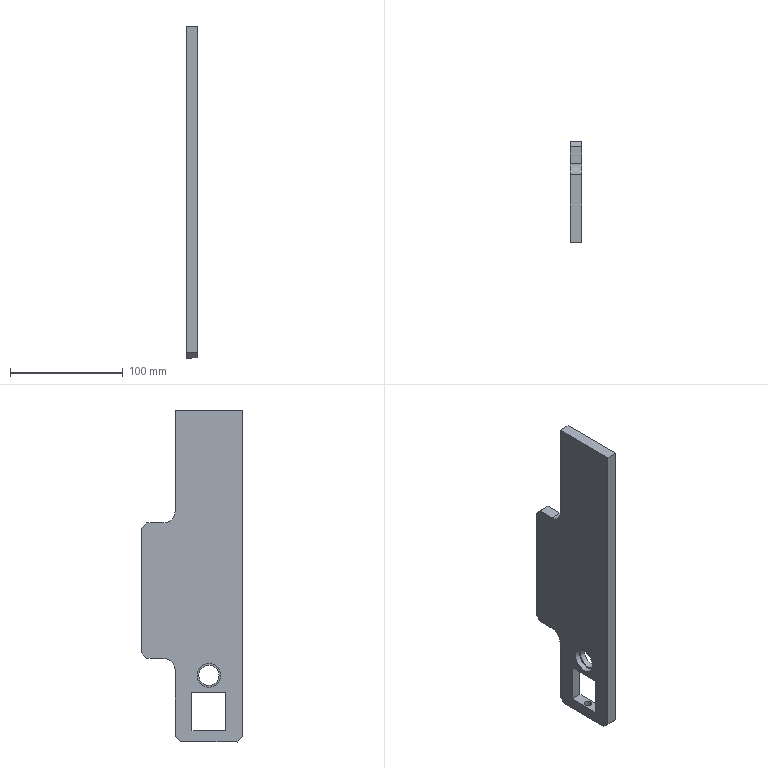Component | SolidWorks | DriveAxis-1_SupportPlate3-1 | 1 solid | 33 faces | box 10 x 90 x 294 mm | volume 198561 mm3 | plane 21 | cylinder 12 | commonest cylinder face diameters 8 x4 6.8 x2 18 x2 21 x2 20 x2
build123d program:
from build123d import *

# Parameters (mm, degrees)
SKETCH1_W             = 60
SKETCH1_H             = 300
BOSS_EXTRUDE1_DEPTH   = 10
SKETCH2_R             = 10.5
CUT_EXTRUDE1_DEPTH    = 5
SKETCH3_R             = 9
CUT_EXTRUDE2_DEPTH    = 306.982
SKETCH4_W             = 30
SKETCH4_H             = 50
CUT_EXTRUDE3_DEPTH    = 307.105
SKETCH5_R             = 4
CUT_EXTRUDE4_DEPTH    = 2
SKETCH6_W             = 30
SKETCH6_H             = 16
BOSS_EXTRUDE2_DEPTH   = 10
SKETCH7_W             = 74.928
SKETCH7_H             = 16.817
CUT_EXTRUDE5_DEPTH    = 307.105
CHAMFER1_SIZE         = 5
M8_TAPPED_HOLE1_D     = 6.8
M8_TAPPED_HOLE1_DEPTH = 19.75
M8_TAPPED_HOLE1_TIP   = 2.043
SKETCH11_W            = 10
SKETCH11_H            = 120
BOSS_EXTRUDE3_DEPTH   = 30
CHAMFER2_SIZE         = 5
FILLET1_R             = 10


with BuildPart() as part:
    # Sketch1 → Boss-Extrude1 (new body)
    with BuildSketch(Plane.XY):
        with Locations((30, -150)):
            Rectangle(SKETCH1_W, SKETCH1_H)
    extrude(amount=BOSS_EXTRUDE1_DEPTH)

    # Sketch2 → Cut-Extrude1 (cut)
    with BuildSketch(Plane.XY.offset(10)):
        with Locations((30, -25)):
            Circle(SKETCH2_R)
        with Locations((30, -65)):
            Circle(SKETCH2_R)
    extrude(amount=-CUT_EXTRUDE1_DEPTH, mode=Mode.SUBTRACT)

    # Sketch3 → Cut-Extrude2 (cut, through all)
    with BuildSketch(Plane.XY.offset(5)):
        with Locations((30, -25)):
            Circle(SKETCH3_R)
        with Locations((30, -65)):
            Circle(SKETCH3_R)
    extrude(amount=-CUT_EXTRUDE2_DEPTH, mode=Mode.SUBTRACT)

    # Sketch4 → Cut-Extrude3 (cut, through all)
    with BuildSketch(Plane.XY.offset(10)):
        with Locations((30, -25)):
            Rectangle(SKETCH4_W, SKETCH4_H)
    extrude(amount=-CUT_EXTRUDE3_DEPTH, mode=Mode.SUBTRACT)

    # Sketch5 → Cut-Extrude4 (cut)
    with BuildSketch(Plane(origin=(0, -50, 0), x_dir=(1, 0, 0), z_dir=(0, 1, 0))):
        with Locations(Location((19.5, -5, 0), (0, 0, 270))):
            Circle(SKETCH5_R)
        with Locations(Location((40.5, -5, 0), (0, 0, 270))):
            Circle(SKETCH5_R)
    extrude(amount=-CUT_EXTRUDE4_DEPTH, mode=Mode.SUBTRACT)

    # Sketch6 → Boss-Extrude2 (add)
    with BuildSketch(Plane(origin=(0, 0, 0), x_dir=(-1, 0, 0), z_dir=(0, 0, -1))):
        with Locations((-30, -8)):
            Rectangle(SKETCH6_W, SKETCH6_H)
    extrude(amount=-BOSS_EXTRUDE2_DEPTH)

    # Sketch7 → Cut-Extrude5 (cut, through all)
    with BuildSketch(Plane.XY.offset(10)):
        with Locations((27.689, 2.409)):
            Rectangle(SKETCH7_W, SKETCH7_H)
    extrude(amount=-CUT_EXTRUDE5_DEPTH, mode=Mode.SUBTRACT)

    # Chamfer1
    chamfer1_edges = [part.edges().sort_by_distance(p)[0] for p in [
        (0, -6, 5),
        (60, -6, 5),
    ]]
    chamfer(chamfer1_edges, length=CHAMFER1_SIZE)

    # M8 Tapped Hole1
    with Locations(Plane(origin=(0, -6, 0), x_dir=(1, 0, 0), z_dir=(0, 1, 0))):
        with Locations((30, -5)):
            Hole(M8_TAPPED_HOLE1_D / 2, depth=M8_TAPPED_HOLE1_DEPTH)
            with Locations((0, 0, -(M8_TAPPED_HOLE1_DEPTH + M8_TAPPED_HOLE1_TIP / 2))):  # 118° drill point
                Cone(0, M8_TAPPED_HOLE1_D / 2, M8_TAPPED_HOLE1_TIP, mode=Mode.SUBTRACT)

    # Sketch11 → Boss-Extrude3 (add)
    with BuildSketch(Plane(origin=(60, 0, 0), x_dir=(0, 0, -1), z_dir=(1, 0, 0))):
        with Locations((-5, -140)):
            Rectangle(SKETCH11_W, SKETCH11_H)
    extrude(amount=BOSS_EXTRUDE3_DEPTH)

    # Chamfer2
    chamfer2_edges = [part.edges().sort_by_distance(p)[0] for p in [
        (90, -200, 5),
        (90, -80, 5),
    ]]
    chamfer(chamfer2_edges, length=CHAMFER2_SIZE)

    # Fillet1
    fillet1_edges = [part.edges().sort_by_distance(p)[0] for p in [
        (60, -200, 5),
        (60, -80, 5),
    ]]
    fillet(fillet1_edges, radius=FILLET1_R)


solid = part.part

# Placed as in the assembly
solid = solid.moved(Location((869, -60, -207.268), (-90, -90, 0)))
STEP:
#1=CARTESIAN_POINT('',(33.882,-1.181,-7.53));
#2=VERTEX_POINT('',#1);
#3=CARTESIAN_POINT('',(34.15,-1.181,-7.53));
#4=VERTEX_POINT('',#3);
#5=CARTESIAN_POINT('',(34.016,-1.181,-7.53));
#6=DIRECTION('',(-0.,-0.,1.));
#7=DIRECTION('',(1.,0.,0.));
#8=AXIS2_PLACEMENT_3D('',#5,#6,#7);
#9=CIRCLE('',#8,0.1339);
#10=EDGE_CURVE('',#2,#4,#9,.T.);
#11=ORIENTED_EDGE('',*,*,#10,.T.);
#12=CARTESIAN_POINT('',(34.15,-1.181,-7.924));
#13=VERTEX_POINT('',#12);
#14=CARTESIAN_POINT('',(34.15,-1.181,-7.924));
#15=DIRECTION('',(0.,0.,-1.));
#16=VECTOR('',#15,39.37);
#17=LINE('',#14,#16);
#18=EDGE_CURVE('',#4,#13,#17,.T.);
#19=ORIENTED_EDGE('',*,*,#18,.T.);
#20=CARTESIAN_POINT('',(33.882,-1.181,-7.924));
#21=VERTEX_POINT('',#20);
#22=CARTESIAN_POINT('',(34.016,-1.181,-7.924));
#23=DIRECTION('',(0.,0.,-1.));
#24=DIRECTION('',(-1.,0.,-0.));
#25=AXIS2_PLACEMENT_3D('',#22,#23,#24);
#26=CIRCLE('',#25,0.1339);
#27=EDGE_CURVE('',#13,#21,#26,.T.);
#28=ORIENTED_EDGE('',*,*,#27,.T.);
#29=CARTESIAN_POINT('',(33.882,-1.181,-7.924));
#30=DIRECTION('',(0.,0.,-1.));
#31=VECTOR('',#30,39.37);
#32=LINE('',#29,#31);
#33=EDGE_CURVE('',#2,#21,#32,.T.);
#34=ORIENTED_EDGE('',*,*,#33,.F.);
#35=EDGE_LOOP('',(#11,#19,#28,#34));
#36=FACE_OUTER_BOUND('',#35,.T.);
#37=CARTESIAN_POINT('',(34.016,-1.181,-7.924));
#38=DIRECTION('',(0.,0.,-1.));
#39=DIRECTION('',(-1.,0.,-0.));
#40=AXIS2_PLACEMENT_3D('',#37,#38,#39);
#41=CYLINDRICAL_SURFACE('',#40,0.1339);
#42=ADVANCED_FACE('',(#36),#41,.F.);
#43=CARTESIAN_POINT('',(34.173,-0.7677,-6.113));
#44=VERTEX_POINT('',#43);
#45=CARTESIAN_POINT('',(33.858,-0.7677,-6.113));
#46=VERTEX_POINT('',#45);
#47=CARTESIAN_POINT('',(34.016,-0.7677,-6.113));
#48=DIRECTION('',(0.,0.,-1.));
#49=DIRECTION('',(-1.,0.,-0.));
#50=AXIS2_PLACEMENT_3D('',#47,#48,#49);
#51=CIRCLE('',#50,0.1575);
#52=EDGE_CURVE('',#44,#46,#51,.T.);
#53=ORIENTED_EDGE('',*,*,#52,.F.);
#54=CARTESIAN_POINT('',(34.173,-0.7677,-6.192));
#55=VERTEX_POINT('',#54);
#56=CARTESIAN_POINT('',(34.173,-0.7677,-6.113));
#57=DIRECTION('',(0.,0.,-1.));
#58=VECTOR('',#57,39.37);
#59=LINE('',#56,#58);
#60=EDGE_CURVE('',#44,#55,#59,.T.);
#61=ORIENTED_EDGE('',*,*,#60,.T.);
#62=CARTESIAN_POINT('',(33.858,-0.7677,-6.192));
#63=VERTEX_POINT('',#62);
#64=CARTESIAN_POINT('',(34.016,-0.7677,-6.192));
#65=DIRECTION('',(0.,0.,-1.));
#66=DIRECTION('',(-1.,0.,-0.));
#67=AXIS2_PLACEMENT_3D('',#64,#65,#66);
#68=CIRCLE('',#67,0.1575);
#69=EDGE_CURVE('',#55,#63,#68,.T.);
#70=ORIENTED_EDGE('',*,*,#69,.T.);
#71=CARTESIAN_POINT('',(33.858,-0.7677,-6.113));
#72=DIRECTION('',(0.,0.,-1.));
#73=VECTOR('',#72,39.37);
#74=LINE('',#71,#73);
#75=EDGE_CURVE('',#46,#63,#74,.T.);
#76=ORIENTED_EDGE('',*,*,#75,.F.);
#77=EDGE_LOOP('',(#53,#61,#70,#76));
#78=FACE_OUTER_BOUND('',#77,.T.);
#79=CARTESIAN_POINT('',(34.016,-0.7677,-6.113));
#80=DIRECTION('',(0.,0.,-1.));
#81=DIRECTION('',(-1.,0.,-0.));
#82=AXIS2_PLACEMENT_3D('',#79,#80,#81);
#83=CYLINDRICAL_SURFACE('',#82,0.1575);
#84=ADVANCED_FACE('',(#78),#83,.F.);
#85=CARTESIAN_POINT('',(34.173,-1.594,-6.113));
#86=VERTEX_POINT('',#85);
#87=CARTESIAN_POINT('',(33.858,-1.594,-6.113));
#88=VERTEX_POINT('',#87);
#89=CARTESIAN_POINT('',(34.016,-1.594,-6.113));
#90=DIRECTION('',(0.,0.,-1.));
#91=DIRECTION('',(-1.,0.,-0.));
#92=AXIS2_PLACEMENT_3D('',#89,#90,#91);
#93=CIRCLE('',#92,0.1575);
#94=EDGE_CURVE('',#86,#88,#93,.T.);
#95=ORIENTED_EDGE('',*,*,#94,.F.);
#96=CARTESIAN_POINT('',(34.173,-1.594,-6.192));
#97=VERTEX_POINT('',#96);
#98=CARTESIAN_POINT('',(34.173,-1.594,-6.113));
#99=DIRECTION('',(0.,0.,-1.));
#100=VECTOR('',#99,39.37);
#101=LINE('',#98,#100);
#102=EDGE_CURVE('',#86,#97,#101,.T.);
#103=ORIENTED_EDGE('',*,*,#102,.T.);
#104=CARTESIAN_POINT('',(33.858,-1.594,-6.192));
#105=VERTEX_POINT('',#104);
#106=CARTESIAN_POINT('',(34.016,-1.594,-6.192));
#107=DIRECTION('',(0.,0.,-1.));
#108=DIRECTION('',(-1.,0.,-0.));
#109=AXIS2_PLACEMENT_3D('',#106,#107,#108);
#110=CIRCLE('',#109,0.1575);
#111=EDGE_CURVE('',#97,#105,#110,.T.);
#112=ORIENTED_EDGE('',*,*,#111,.T.);
#113=CARTESIAN_POINT('',(33.858,-1.594,-6.113));
#114=DIRECTION('',(0.,0.,-1.));
#115=VECTOR('',#114,39.37);
#116=LINE('',#113,#115);
#117=EDGE_CURVE('',#88,#105,#116,.T.);
#118=ORIENTED_EDGE('',*,*,#117,.F.);
#119=EDGE_LOOP('',(#95,#103,#112,#118));
#120=FACE_OUTER_BOUND('',#119,.T.);
#121=CARTESIAN_POINT('',(34.016,-1.594,-6.113));
#122=DIRECTION('',(0.,0.,-1.));
#123=DIRECTION('',(-1.,0.,-0.));
#124=AXIS2_PLACEMENT_3D('',#121,#122,#123);
#125=CYLINDRICAL_SURFACE('',#124,0.1575);
#126=ADVANCED_FACE('',(#120),#125,.F.);
#127=CARTESIAN_POINT('',(34.213,-1.535,-5.601));
#128=VERTEX_POINT('',#127);
#129=CARTESIAN_POINT('',(34.213,-0.8268,-5.601));
#130=VERTEX_POINT('',#129);
#131=CARTESIAN_POINT('',(34.213,-1.181,-5.601));
#132=DIRECTION('',(-1.,-0.,-0.));
#133=DIRECTION('',(0.,1.,0.));
#134=AXIS2_PLACEMENT_3D('',#131,#132,#133);
#135=CIRCLE('',#134,0.3543);
#136=EDGE_CURVE('',#128,#130,#135,.T.);
#137=ORIENTED_EDGE('',*,*,#136,.F.);
#138=CARTESIAN_POINT('',(34.016,-1.535,-5.601));
#139=VERTEX_POINT('',#138);
#140=CARTESIAN_POINT('',(34.213,-1.535,-5.601));
#141=DIRECTION('',(-1.,-0.,-0.));
#142=VECTOR('',#141,39.37);
#143=LINE('',#140,#142);
#144=EDGE_CURVE('',#128,#139,#143,.T.);
#145=ORIENTED_EDGE('',*,*,#144,.T.);
#146=CARTESIAN_POINT('',(34.016,-0.8268,-5.601));
#147=VERTEX_POINT('',#146);
#148=CARTESIAN_POINT('',(34.016,-1.181,-5.601));
#149=DIRECTION('',(-1.,-0.,-0.));
#150=DIRECTION('',(0.,1.,0.));
#151=AXIS2_PLACEMENT_3D('',#148,#149,#150);
#152=CIRCLE('',#151,0.3543);
#153=EDGE_CURVE('',#139,#147,#152,.T.);
#154=ORIENTED_EDGE('',*,*,#153,.T.);
#155=CARTESIAN_POINT('',(34.213,-0.8268,-5.601));
#156=DIRECTION('',(-1.,-0.,-0.));
#157=VECTOR('',#156,39.37);
#158=LINE('',#155,#157);
#159=EDGE_CURVE('',#130,#147,#158,.T.);
#160=ORIENTED_EDGE('',*,*,#159,.F.);
#161=EDGE_LOOP('',(#137,#145,#154,#160));
#162=FACE_OUTER_BOUND('',#161,.T.);
#163=CARTESIAN_POINT('',(34.213,-1.181,-5.601));
#164=DIRECTION('',(-1.,-0.,-0.));
#165=DIRECTION('',(0.,1.,0.));
#166=AXIS2_PLACEMENT_3D('',#163,#164,#165);
#167=CYLINDRICAL_SURFACE('',#166,0.3543);
#168=ADVANCED_FACE('',(#162),#167,.F.);
#169=CARTESIAN_POINT('',(34.016,-1.594,-5.601));
#170=VERTEX_POINT('',#169);
#171=CARTESIAN_POINT('',(34.016,-0.7677,-5.601));
#172=VERTEX_POINT('',#171);
#173=CARTESIAN_POINT('',(34.016,-1.181,-5.601));
#174=DIRECTION('',(-1.,-0.,-0.));
#175=DIRECTION('',(0.,1.,0.));
#176=AXIS2_PLACEMENT_3D('',#173,#174,#175);
#177=CIRCLE('',#176,0.4134);
#178=EDGE_CURVE('',#170,#172,#177,.T.);
#179=ORIENTED_EDGE('',*,*,#178,.F.);
#180=CARTESIAN_POINT('',(33.819,-1.594,-5.601));
#181=VERTEX_POINT('',#180);
#182=CARTESIAN_POINT('',(34.016,-1.594,-5.601));
#183=DIRECTION('',(-1.,-0.,-0.));
#184=VECTOR('',#183,39.37);
#185=LINE('',#182,#184);
#186=EDGE_CURVE('',#170,#181,#185,.T.);
#187=ORIENTED_EDGE('',*,*,#186,.T.);
#188=CARTESIAN_POINT('',(33.819,-0.7677,-5.601));
#189=VERTEX_POINT('',#188);
#190=CARTESIAN_POINT('',(33.819,-1.181,-5.601));
#191=DIRECTION('',(-1.,-0.,-0.));
#192=DIRECTION('',(0.,1.,0.));
#193=AXIS2_PLACEMENT_3D('',#190,#191,#192);
#194=CIRCLE('',#193,0.4134);
#195=EDGE_CURVE('',#181,#189,#194,.T.);
#196=ORIENTED_EDGE('',*,*,#195,.T.);
#197=CARTESIAN_POINT('',(34.016,-0.7677,-5.601));
#198=DIRECTION('',(-1.,-0.,-0.));
#199=VECTOR('',#198,39.37);
#200=LINE('',#197,#199);
#201=EDGE_CURVE('',#172,#189,#200,.T.);
#202=ORIENTED_EDGE('',*,*,#201,.F.);
#203=EDGE_LOOP('',(#179,#187,#196,#202));
#204=FACE_OUTER_BOUND('',#203,.T.);
#205=CARTESIAN_POINT('',(34.016,-1.181,-5.601));
#206=DIRECTION('',(-1.,-0.,-0.));
#207=DIRECTION('',(0.,1.,0.));
#208=AXIS2_PLACEMENT_3D('',#205,#206,#207);
#209=CYLINDRICAL_SURFACE('',#208,0.4134);
#210=ADVANCED_FACE('',(#204),#209,.F.);
#211=CARTESIAN_POINT('',(33.819,-0.,-5.404));
#212=VERTEX_POINT('',#211);
#213=CARTESIAN_POINT('',(33.819,0.,-7.727));
#214=VERTEX_POINT('',#213);
#215=CARTESIAN_POINT('',(33.819,0.,-8.16));
#216=DIRECTION('',(0.,0.,-1.));
#217=VECTOR('',#216,39.37);
#218=LINE('',#215,#217);
#219=EDGE_CURVE('',#212,#214,#218,.T.);
#220=ORIENTED_EDGE('',*,*,#219,.F.);
#221=CARTESIAN_POINT('',(34.213,-0.,-5.404));
#222=VERTEX_POINT('',#221);
#223=CARTESIAN_POINT('',(34.213,-0.,-5.404));
#224=DIRECTION('',(1.,0.,0.));
#225=VECTOR('',#224,39.37);
#226=LINE('',#223,#225);
#227=EDGE_CURVE('',#212,#222,#226,.T.);
#228=ORIENTED_EDGE('',*,*,#227,.T.);
#229=CARTESIAN_POINT('',(34.213,0.,-7.727));
#230=VERTEX_POINT('',#229);
#231=CARTESIAN_POINT('',(34.213,0.,-8.16));
#232=DIRECTION('',(0.,0.,-1.));
#233=VECTOR('',#232,39.37);
#234=LINE('',#231,#233);
#235=EDGE_CURVE('',#222,#230,#234,.T.);
#236=ORIENTED_EDGE('',*,*,#235,.T.);
#237=CARTESIAN_POINT('',(33.819,0.,-7.727));
#238=DIRECTION('',(-1.,-0.,-0.));
#239=VECTOR('',#238,39.37);
#240=LINE('',#237,#239);
#241=EDGE_CURVE('',#230,#214,#240,.T.);
#242=ORIENTED_EDGE('',*,*,#241,.T.);
#243=EDGE_LOOP('',(#220,#228,#236,#242));
#244=FACE_OUTER_BOUND('',#243,.T.);
#245=CARTESIAN_POINT('',(33.819,0.,-8.16));
#246=DIRECTION('',(0.,-1.,-0.));
#247=DIRECTION('',(-0.,-0.,1.));
#248=AXIS2_PLACEMENT_3D('',#245,#246,#247);
#249=PLANE('',#248);
#250=ADVANCED_FACE('',(#244),#249,.F.);
#251=CARTESIAN_POINT('',(34.213,-0.,3.651));
#252=VERTEX_POINT('',#251);
#253=CARTESIAN_POINT('',(34.213,-0.,0.1076));
#254=VERTEX_POINT('',#253);
#255=CARTESIAN_POINT('',(34.213,0.,-8.16));
#256=DIRECTION('',(0.,0.,-1.));
#257=VECTOR('',#256,39.37);
#258=LINE('',#255,#257);
#259=EDGE_CURVE('',#252,#254,#258,.T.);
#260=ORIENTED_EDGE('',*,*,#259,.T.);
#261=CARTESIAN_POINT('',(33.819,-0.,0.1076));
#262=VERTEX_POINT('',#261);
#263=CARTESIAN_POINT('',(33.819,-0.,0.1076));
#264=DIRECTION('',(-1.,-0.,-0.));
#265=VECTOR('',#264,39.37);
#266=LINE('',#263,#265);
#267=EDGE_CURVE('',#254,#262,#266,.T.);
#268=ORIENTED_EDGE('',*,*,#267,.T.);
#269=CARTESIAN_POINT('',(33.819,-0.,3.651));
#270=VERTEX_POINT('',#269);
#271=CARTESIAN_POINT('',(33.819,0.,-8.16));
#272=DIRECTION('',(0.,0.,-1.));
#273=VECTOR('',#272,39.37);
#274=LINE('',#271,#273);
#275=EDGE_CURVE('',#270,#262,#274,.T.);
#276=ORIENTED_EDGE('',*,*,#275,.F.);
#277=CARTESIAN_POINT('',(33.819,-0.,3.651));
#278=DIRECTION('',(1.,0.,0.));
#279=VECTOR('',#278,39.37);
#280=LINE('',#277,#279);
#281=EDGE_CURVE('',#270,#252,#280,.T.);
#282=ORIENTED_EDGE('',*,*,#281,.T.);
#283=EDGE_LOOP('',(#260,#268,#276,#282));
#284=FACE_OUTER_BOUND('',#283,.T.);
#285=CARTESIAN_POINT('',(33.819,0.,-8.16));
#286=DIRECTION('',(0.,-1.,-0.));
#287=DIRECTION('',(-0.,-0.,1.));
#288=AXIS2_PLACEMENT_3D('',#285,#286,#287);
#289=PLANE('',#288);
#290=ADVANCED_FACE('',(#284),#289,.F.);
#291=CARTESIAN_POINT('',(33.819,-2.362,-7.727));
#292=VERTEX_POINT('',#291);
#293=CARTESIAN_POINT('',(33.819,-2.362,3.651));
#294=VERTEX_POINT('',#293);
#295=CARTESIAN_POINT('',(33.819,-2.362,-8.16));
#296=DIRECTION('',(-0.,-0.,1.));
#297=VECTOR('',#296,39.37);
#298=LINE('',#295,#297);
#299=EDGE_CURVE('',#292,#294,#298,.T.);
#300=ORIENTED_EDGE('',*,*,#299,.F.);
#301=CARTESIAN_POINT('',(34.213,-2.362,-7.727));
#302=VERTEX_POINT('',#301);
#303=CARTESIAN_POINT('',(33.819,-2.362,-7.727));
#304=DIRECTION('',(1.,0.,0.));
#305=VECTOR('',#304,39.37);
#306=LINE('',#303,#305);
#307=EDGE_CURVE('',#292,#302,#306,.T.);
#308=ORIENTED_EDGE('',*,*,#307,.T.);
#309=CARTESIAN_POINT('',(34.213,-2.362,3.651));
#310=VERTEX_POINT('',#309);
#311=CARTESIAN_POINT('',(34.213,-2.362,-8.16));
#312=DIRECTION('',(-0.,-0.,1.));
#313=VECTOR('',#312,39.37);
#314=LINE('',#311,#313);
#315=EDGE_CURVE('',#302,#310,#314,.T.);
#316=ORIENTED_EDGE('',*,*,#315,.T.);
#317=CARTESIAN_POINT('',(33.819,-2.362,3.651));
#318=DIRECTION('',(1.,0.,0.));
#319=VECTOR('',#318,39.37);
#320=LINE('',#317,#319);
#321=EDGE_CURVE('',#294,#310,#320,.T.);
#322=ORIENTED_EDGE('',*,*,#321,.F.);
#323=EDGE_LOOP('',(#300,#308,#316,#322));
#324=FACE_OUTER_BOUND('',#323,.T.);
#325=CARTESIAN_POINT('',(33.819,-2.362,-8.16));
#326=DIRECTION('',(-0.,1.,0.));
#327=DIRECTION('',(0.,0.,-1.));
#328=AXIS2_PLACEMENT_3D('',#325,#326,#327);
#329=PLANE('',#328);
#330=ADVANCED_FACE('',(#324),#329,.F.);
#331=CARTESIAN_POINT('',(34.213,-2.362,3.651));
#332=DIRECTION('',(-0.,1.,0.));
#333=VECTOR('',#332,39.37);
#334=LINE('',#331,#333);
#335=EDGE_CURVE('',#310,#252,#334,.T.);
#336=ORIENTED_EDGE('',*,*,#335,.T.);
#337=ORIENTED_EDGE('',*,*,#281,.F.);
#338=CARTESIAN_POINT('',(33.819,-2.362,3.651));
#339=DIRECTION('',(-0.,1.,0.));
#340=VECTOR('',#339,39.37);
#341=LINE('',#338,#340);
#342=EDGE_CURVE('',#294,#270,#341,.T.);
#343=ORIENTED_EDGE('',*,*,#342,.F.);
#344=ORIENTED_EDGE('',*,*,#321,.T.);
#345=EDGE_LOOP('',(#336,#337,#343,#344));
#346=FACE_OUTER_BOUND('',#345,.T.);
#347=CARTESIAN_POINT('',(33.819,-2.362,3.651));
#348=DIRECTION('',(0.,0.,-1.));
#349=DIRECTION('',(-1.,-0.,-0.));
#350=AXIS2_PLACEMENT_3D('',#347,#348,#349);
#351=PLANE('',#350);
#352=ADVANCED_FACE('',(#346),#351,.F.);
#353=CARTESIAN_POINT('',(33.819,0.9843,-0.2861));
#354=VERTEX_POINT('',#353);
#355=CARTESIAN_POINT('',(33.819,0.3937,-0.2861));
#356=VERTEX_POINT('',#355);
#357=CARTESIAN_POINT('',(33.819,1.181,-0.2861));
#358=DIRECTION('',(0.,-1.,-0.));
#359=VECTOR('',#358,39.37);
#360=LINE('',#357,#359);
#361=EDGE_CURVE('',#354,#356,#360,.T.);
#362=ORIENTED_EDGE('',*,*,#361,.F.);
#363=CARTESIAN_POINT('',(33.819,1.181,-0.483));
#364=VERTEX_POINT('',#363);
#365=CARTESIAN_POINT('',(33.819,3.248,-2.55));
#366=DIRECTION('',(0.,0.7071,-0.7071));
#367=VECTOR('',#366,39.37);
#368=LINE('',#365,#367);
#369=EDGE_CURVE('',#354,#364,#368,.T.);
#370=ORIENTED_EDGE('',*,*,#369,.T.);
#371=CARTESIAN_POINT('',(33.819,1.181,-4.814));
#372=VERTEX_POINT('',#371);
#373=CARTESIAN_POINT('',(33.819,1.181,-5.011));
#374=DIRECTION('',(-0.,-0.,1.));
#375=VECTOR('',#374,39.37);
#376=LINE('',#373,#375);
#377=EDGE_CURVE('',#372,#364,#376,.T.);
#378=ORIENTED_EDGE('',*,*,#377,.F.);
#379=CARTESIAN_POINT('',(33.819,0.9843,-5.011));
#380=VERTEX_POINT('',#379);
#381=CARTESIAN_POINT('',(33.819,-2.264,-8.259));
#382=DIRECTION('',(0.,-0.7071,-0.7071));
#383=VECTOR('',#382,39.37);
#384=LINE('',#381,#383);
#385=EDGE_CURVE('',#372,#380,#384,.T.);
#386=ORIENTED_EDGE('',*,*,#385,.T.);
#387=CARTESIAN_POINT('',(33.819,0.3937,-5.011));
#388=VERTEX_POINT('',#387);
#389=CARTESIAN_POINT('',(33.819,1.181,-5.011));
#390=DIRECTION('',(0.,-1.,-0.));
#391=VECTOR('',#390,39.37);
#392=LINE('',#389,#391);
#393=EDGE_CURVE('',#380,#388,#392,.T.);
#394=ORIENTED_EDGE('',*,*,#393,.T.);
#395=CARTESIAN_POINT('',(33.819,0.3937,-5.404));
#396=DIRECTION('',(1.,0.,0.));
#397=DIRECTION('',(0.,1.,0.));
#398=AXIS2_PLACEMENT_3D('',#395,#396,#397);
#399=CIRCLE('',#398,0.3937);
#400=EDGE_CURVE('',#388,#212,#399,.T.);
#401=ORIENTED_EDGE('',*,*,#400,.T.);
#402=ORIENTED_EDGE('',*,*,#219,.T.);
#403=CARTESIAN_POINT('',(33.819,-0.1969,-7.924));
#404=VERTEX_POINT('',#403);
#405=CARTESIAN_POINT('',(33.819,-1.398,-9.125));
#406=DIRECTION('',(0.,-0.7071,-0.7071));
#407=VECTOR('',#406,39.37);
#408=LINE('',#405,#407);
#409=EDGE_CURVE('',#214,#404,#408,.T.);
#410=ORIENTED_EDGE('',*,*,#409,.T.);
#411=CARTESIAN_POINT('',(33.819,-2.165,-7.924));
#412=VERTEX_POINT('',#411);
#413=CARTESIAN_POINT('',(33.819,-2.747,-7.924));
#414=DIRECTION('',(-0.,1.,0.));
#415=VECTOR('',#414,39.37);
#416=LINE('',#413,#415);
#417=EDGE_CURVE('',#412,#404,#416,.T.);
#418=ORIENTED_EDGE('',*,*,#417,.F.);
#419=CARTESIAN_POINT('',(33.819,-2.146,-7.944));
#420=DIRECTION('',(-0.,-0.7071,0.7071));
#421=VECTOR('',#420,39.37);
#422=LINE('',#419,#421);
#423=EDGE_CURVE('',#412,#292,#422,.T.);
#424=ORIENTED_EDGE('',*,*,#423,.T.);
#425=ORIENTED_EDGE('',*,*,#299,.T.);
#426=ORIENTED_EDGE('',*,*,#342,.T.);
#427=ORIENTED_EDGE('',*,*,#275,.T.);
#428=CARTESIAN_POINT('',(33.819,0.3937,0.1076));
#429=DIRECTION('',(1.,0.,0.));
#430=DIRECTION('',(0.,1.,0.));
#431=AXIS2_PLACEMENT_3D('',#428,#429,#430);
#432=CIRCLE('',#431,0.3937);
#433=EDGE_CURVE('',#262,#356,#432,.T.);
#434=ORIENTED_EDGE('',*,*,#433,.T.);
#435=EDGE_LOOP('',(#362,#370,#378,#386,#394,#401,#402,#410,#418,#424,#425,#426,#427,#434));
#436=FACE_OUTER_BOUND('',#435,.T.);
#437=CARTESIAN_POINT('',(33.819,-1.772,-7.53));
#438=VERTEX_POINT('',#437);
#439=CARTESIAN_POINT('',(33.819,-1.772,-6.192));
#440=VERTEX_POINT('',#439);
#441=CARTESIAN_POINT('',(33.819,-1.772,-8.16));
#442=DIRECTION('',(-0.,-0.,1.));
#443=VECTOR('',#442,39.37);
#444=LINE('',#441,#443);
#445=EDGE_CURVE('',#438,#440,#444,.T.);
#446=ORIENTED_EDGE('',*,*,#445,.F.);
#447=CARTESIAN_POINT('',(33.819,-0.5906,-7.53));
#448=VERTEX_POINT('',#447);
#449=CARTESIAN_POINT('',(33.819,-0.5906,-7.53));
#450=DIRECTION('',(0.,-1.,-0.));
#451=VECTOR('',#450,39.37);
#452=LINE('',#449,#451);
#453=EDGE_CURVE('',#448,#438,#452,.T.);
#454=ORIENTED_EDGE('',*,*,#453,.F.);
#455=CARTESIAN_POINT('',(33.819,-0.5906,-6.192));
#456=VERTEX_POINT('',#455);
#457=CARTESIAN_POINT('',(33.819,-0.5906,-8.16));
#458=DIRECTION('',(0.,0.,-1.));
#459=VECTOR('',#458,39.37);
#460=LINE('',#457,#459);
#461=EDGE_CURVE('',#456,#448,#460,.T.);
#462=ORIENTED_EDGE('',*,*,#461,.F.);
#463=CARTESIAN_POINT('',(33.819,-1.772,-6.192));
#464=DIRECTION('',(-0.,1.,0.));
#465=VECTOR('',#464,39.37);
#466=LINE('',#463,#465);
#467=EDGE_CURVE('',#440,#456,#466,.T.);
#468=ORIENTED_EDGE('',*,*,#467,.F.);
#469=EDGE_LOOP('',(#446,#454,#462,#468));
#470=FACE_BOUND('',#469,.T.);
#471=CARTESIAN_POINT('',(33.819,-1.181,-5.601));
#472=DIRECTION('',(-1.,-0.,-0.));
#473=DIRECTION('',(0.,1.,0.));
#474=AXIS2_PLACEMENT_3D('',#471,#472,#473);
#475=CIRCLE('',#474,0.4134);
#476=EDGE_CURVE('',#189,#181,#475,.T.);
#477=ORIENTED_EDGE('',*,*,#476,.F.);
#478=ORIENTED_EDGE('',*,*,#195,.F.);
#479=EDGE_LOOP('',(#477,#478));
#480=FACE_BOUND('',#479,.T.);
#481=CARTESIAN_POINT('',(33.819,-2.362,-8.16));
#482=DIRECTION('',(-1.,-0.,-0.));
#483=DIRECTION('',(-0.,1.,0.));
#484=AXIS2_PLACEMENT_3D('',#481,#482,#483);
#485=PLANE('',#484);
#486=ADVANCED_FACE('',(#436,#470,#480),#485,.T.);
#487=CARTESIAN_POINT('',(34.213,-0.5906,-7.53));
#488=VERTEX_POINT('',#487);
#489=CARTESIAN_POINT('',(34.213,-1.772,-7.53));
#490=VERTEX_POINT('',#489);
#491=CARTESIAN_POINT('',(34.213,-0.5906,-7.53));
#492=DIRECTION('',(0.,-1.,-0.));
#493=VECTOR('',#492,39.37);
#494=LINE('',#491,#493);
#495=EDGE_CURVE('',#488,#490,#494,.T.);
#496=ORIENTED_EDGE('',*,*,#495,.T.);
#497=CARTESIAN_POINT('',(34.213,-1.772,-6.192));
#498=VERTEX_POINT('',#497);
#499=CARTESIAN_POINT('',(34.213,-1.772,-8.16));
#500=DIRECTION('',(-0.,-0.,1.));
#501=VECTOR('',#500,39.37);
#502=LINE('',#499,#501);
#503=EDGE_CURVE('',#490,#498,#502,.T.);
#504=ORIENTED_EDGE('',*,*,#503,.T.);
#505=CARTESIAN_POINT('',(34.213,-0.5906,-6.192));
#506=VERTEX_POINT('',#505);
#507=CARTESIAN_POINT('',(34.213,-1.772,-6.192));
#508=DIRECTION('',(-0.,1.,0.));
#509=VECTOR('',#508,39.37);
#510=LINE('',#507,#509);
#511=EDGE_CURVE('',#498,#506,#510,.T.);
#512=ORIENTED_EDGE('',*,*,#511,.T.);
#513=CARTESIAN_POINT('',(34.213,-0.5906,-8.16));
#514=DIRECTION('',(0.,0.,-1.));
#515=VECTOR('',#514,39.37);
#516=LINE('',#513,#515);
#517=EDGE_CURVE('',#506,#488,#516,.T.);
#518=ORIENTED_EDGE('',*,*,#517,.T.);
#519=EDGE_LOOP('',(#496,#504,#512,#518));
#520=FACE_BOUND('',#519,.T.);
#521=CARTESIAN_POINT('',(34.213,1.181,-0.483));
#522=VERTEX_POINT('',#521);
#523=CARTESIAN_POINT('',(34.213,1.181,-4.814));
#524=VERTEX_POINT('',#523);
#525=CARTESIAN_POINT('',(34.213,1.181,-5.011));
#526=DIRECTION('',(0.,0.,-1.));
#527=VECTOR('',#526,39.37);
#528=LINE('',#525,#527);
#529=EDGE_CURVE('',#522,#524,#528,.T.);
#530=ORIENTED_EDGE('',*,*,#529,.F.);
#531=CARTESIAN_POINT('',(34.213,0.9843,-0.2861));
#532=VERTEX_POINT('',#531);
#533=CARTESIAN_POINT('',(34.213,1.181,-0.483));
#534=DIRECTION('',(-0.,-0.7071,0.7071));
#535=VECTOR('',#534,39.37);
#536=LINE('',#533,#535);
#537=EDGE_CURVE('',#522,#532,#536,.T.);
#538=ORIENTED_EDGE('',*,*,#537,.T.);
#539=CARTESIAN_POINT('',(34.213,0.3937,-0.2861));
#540=VERTEX_POINT('',#539);
#541=CARTESIAN_POINT('',(34.213,1.181,-0.2861));
#542=DIRECTION('',(0.,-1.,-0.));
#543=VECTOR('',#542,39.37);
#544=LINE('',#541,#543);
#545=EDGE_CURVE('',#532,#540,#544,.T.);
#546=ORIENTED_EDGE('',*,*,#545,.T.);
#547=CARTESIAN_POINT('',(34.213,0.3937,0.1076));
#548=DIRECTION('',(-1.,-0.,-0.));
#549=DIRECTION('',(0.,1.,0.));
#550=AXIS2_PLACEMENT_3D('',#547,#548,#549);
#551=CIRCLE('',#550,0.3937);
#552=EDGE_CURVE('',#540,#254,#551,.T.);
#553=ORIENTED_EDGE('',*,*,#552,.T.);
#554=ORIENTED_EDGE('',*,*,#259,.F.);
#555=ORIENTED_EDGE('',*,*,#335,.F.);
#556=ORIENTED_EDGE('',*,*,#315,.F.);
#557=CARTESIAN_POINT('',(34.213,-2.165,-7.924));
#558=VERTEX_POINT('',#557);
#559=CARTESIAN_POINT('',(34.213,-2.362,-7.727));
#560=DIRECTION('',(0.,0.7071,-0.7071));
#561=VECTOR('',#560,39.37);
#562=LINE('',#559,#561);
#563=EDGE_CURVE('',#302,#558,#562,.T.);
#564=ORIENTED_EDGE('',*,*,#563,.T.);
#565=CARTESIAN_POINT('',(34.213,-0.1969,-7.924));
#566=VERTEX_POINT('',#565);
#567=CARTESIAN_POINT('',(34.213,-2.362,-7.924));
#568=DIRECTION('',(-0.,1.,0.));
#569=VECTOR('',#568,39.37);
#570=LINE('',#567,#569);
#571=EDGE_CURVE('',#558,#566,#570,.T.);
#572=ORIENTED_EDGE('',*,*,#571,.T.);
#573=CARTESIAN_POINT('',(34.213,0.,-7.727));
#574=DIRECTION('',(-0.,0.7071,0.7071));
#575=VECTOR('',#574,39.37);
#576=LINE('',#573,#575);
#577=EDGE_CURVE('',#566,#230,#576,.T.);
#578=ORIENTED_EDGE('',*,*,#577,.T.);
#579=ORIENTED_EDGE('',*,*,#235,.F.);
#580=CARTESIAN_POINT('',(34.213,0.3937,-5.011));
#581=VERTEX_POINT('',#580);
#582=CARTESIAN_POINT('',(34.213,0.3937,-5.404));
#583=DIRECTION('',(-1.,-0.,-0.));
#584=DIRECTION('',(0.,1.,0.));
#585=AXIS2_PLACEMENT_3D('',#582,#583,#584);
#586=CIRCLE('',#585,0.3937);
#587=EDGE_CURVE('',#222,#581,#586,.T.);
#588=ORIENTED_EDGE('',*,*,#587,.T.);
#589=CARTESIAN_POINT('',(34.213,0.9843,-5.011));
#590=VERTEX_POINT('',#589);
#591=CARTESIAN_POINT('',(34.213,1.181,-5.011));
#592=DIRECTION('',(0.,-1.,-0.));
#593=VECTOR('',#592,39.37);
#594=LINE('',#591,#593);
#595=EDGE_CURVE('',#590,#581,#594,.T.);
#596=ORIENTED_EDGE('',*,*,#595,.F.);
#597=CARTESIAN_POINT('',(34.213,1.181,-4.814));
#598=DIRECTION('',(-0.,0.7071,0.7071));
#599=VECTOR('',#598,39.37);
#600=LINE('',#597,#599);
#601=EDGE_CURVE('',#590,#524,#600,.T.);
#602=ORIENTED_EDGE('',*,*,#601,.T.);
#603=EDGE_LOOP('',(#530,#538,#546,#553,#554,#555,#556,#564,#572,#578,#579,#588,#596,#602));
#604=FACE_OUTER_BOUND('',#603,.T.);
#605=CARTESIAN_POINT('',(34.213,-1.181,-5.601));
#606=DIRECTION('',(-1.,-0.,-0.));
#607=DIRECTION('',(0.,1.,0.));
#608=AXIS2_PLACEMENT_3D('',#605,#606,#607);
#609=CIRCLE('',#608,0.3543);
#610=EDGE_CURVE('',#130,#128,#609,.T.);
#611=ORIENTED_EDGE('',*,*,#610,.T.);
#612=ORIENTED_EDGE('',*,*,#136,.T.);
#613=EDGE_LOOP('',(#611,#612));
#614=FACE_BOUND('',#613,.T.);
#615=CARTESIAN_POINT('',(34.213,-2.362,-8.16));
#616=DIRECTION('',(-1.,-0.,-0.));
#617=DIRECTION('',(-0.,1.,0.));
#618=AXIS2_PLACEMENT_3D('',#615,#616,#617);
#619=PLANE('',#618);
#620=ADVANCED_FACE('',(#520,#604,#614),#619,.F.);
#621=ORIENTED_EDGE('',*,*,#186,.F.);
#622=CARTESIAN_POINT('',(34.016,-1.181,-5.601));
#623=DIRECTION('',(-1.,-0.,-0.));
#624=DIRECTION('',(0.,1.,0.));
#625=AXIS2_PLACEMENT_3D('',#622,#623,#624);
#626=CIRCLE('',#625,0.4134);
#627=EDGE_CURVE('',#172,#170,#626,.T.);
#628=ORIENTED_EDGE('',*,*,#627,.F.);
#629=ORIENTED_EDGE('',*,*,#201,.T.);
#630=ORIENTED_EDGE('',*,*,#476,.T.);
#631=EDGE_LOOP('',(#621,#628,#629,#630));
#632=FACE_OUTER_BOUND('',#631,.T.);
#633=CARTESIAN_POINT('',(34.016,-1.181,-5.601));
#634=DIRECTION('',(-1.,-0.,-0.));
#635=DIRECTION('',(0.,1.,0.));
#636=AXIS2_PLACEMENT_3D('',#633,#634,#635);
#637=CYLINDRICAL_SURFACE('',#636,0.4134);
#638=ADVANCED_FACE('',(#632),#637,.F.);
#639=CARTESIAN_POINT('',(34.016,-1.181,-5.601));
#640=DIRECTION('',(-1.,-0.,-0.));
#641=DIRECTION('',(0.,1.,0.));
#642=AXIS2_PLACEMENT_3D('',#639,#640,#641);
#643=CIRCLE('',#642,0.3543);
#644=EDGE_CURVE('',#147,#139,#643,.T.);
#645=ORIENTED_EDGE('',*,*,#644,.F.);
#646=ORIENTED_EDGE('',*,*,#153,.F.);
#647=EDGE_LOOP('',(#645,#646));
#648=FACE_BOUND('',#647,.T.);
#649=ORIENTED_EDGE('',*,*,#627,.T.);
#650=ORIENTED_EDGE('',*,*,#178,.T.);
#651=EDGE_LOOP('',(#649,#650));
#652=FACE_OUTER_BOUND('',#651,.T.);
#653=CARTESIAN_POINT('',(34.016,-1.181,-5.601));
#654=DIRECTION('',(-1.,-0.,-0.));
#655=DIRECTION('',(-0.,1.,0.));
#656=AXIS2_PLACEMENT_3D('',#653,#654,#655);
#657=PLANE('',#656);
#658=ADVANCED_FACE('',(#648,#652),#657,.T.);
#659=ORIENTED_EDGE('',*,*,#144,.F.);
#660=ORIENTED_EDGE('',*,*,#610,.F.);
#661=ORIENTED_EDGE('',*,*,#159,.T.);
#662=ORIENTED_EDGE('',*,*,#644,.T.);
#663=EDGE_LOOP('',(#659,#660,#661,#662));
#664=FACE_OUTER_BOUND('',#663,.T.);
#665=CARTESIAN_POINT('',(34.213,-1.181,-5.601));
#666=DIRECTION('',(-1.,-0.,-0.));
#667=DIRECTION('',(0.,1.,0.));
#668=AXIS2_PLACEMENT_3D('',#665,#666,#667);
#669=CYLINDRICAL_SURFACE('',#668,0.3543);
#670=ADVANCED_FACE('',(#664),#669,.F.);
#671=ORIENTED_EDGE('',*,*,#503,.F.);
#672=CARTESIAN_POINT('',(32.48,-1.772,-7.53));
#673=DIRECTION('',(1.,0.,0.));
#674=VECTOR('',#673,39.37);
#675=LINE('',#672,#674);
#676=EDGE_CURVE('',#438,#490,#675,.T.);
#677=ORIENTED_EDGE('',*,*,#676,.F.);
#678=ORIENTED_EDGE('',*,*,#445,.T.);
#679=CARTESIAN_POINT('',(34.213,-1.772,-6.192));
#680=DIRECTION('',(-1.,-0.,-0.));
#681=VECTOR('',#680,39.37);
#682=LINE('',#679,#681);
#683=EDGE_CURVE('',#498,#440,#682,.T.);
#684=ORIENTED_EDGE('',*,*,#683,.F.);
#685=EDGE_LOOP('',(#671,#677,#678,#684));
#686=FACE_OUTER_BOUND('',#685,.T.);
#687=CARTESIAN_POINT('',(34.213,-1.772,-8.16));
#688=DIRECTION('',(0.,-1.,-0.));
#689=DIRECTION('',(-0.,-0.,1.));
#690=AXIS2_PLACEMENT_3D('',#687,#688,#689);
#691=PLANE('',#690);
#692=ADVANCED_FACE('',(#686),#691,.F.);
#693=ORIENTED_EDGE('',*,*,#461,.T.);
#694=CARTESIAN_POINT('',(32.48,-0.5906,-7.53));
#695=DIRECTION('',(1.,0.,0.));
#696=VECTOR('',#695,39.37);
#697=LINE('',#694,#696);
#698=EDGE_CURVE('',#448,#488,#697,.T.);
#699=ORIENTED_EDGE('',*,*,#698,.T.);
#700=ORIENTED_EDGE('',*,*,#517,.F.);
#701=CARTESIAN_POINT('',(34.213,-0.5906,-6.192));
#702=DIRECTION('',(-1.,-0.,-0.));
#703=VECTOR('',#702,39.37);
#704=LINE('',#701,#703);
#705=EDGE_CURVE('',#506,#456,#704,.T.);
#706=ORIENTED_EDGE('',*,*,#705,.T.);
#707=EDGE_LOOP('',(#693,#699,#700,#706));
#708=FACE_OUTER_BOUND('',#707,.T.);
#709=CARTESIAN_POINT('',(34.213,-0.5906,-8.16));
#710=DIRECTION('',(-0.,1.,0.));
#711=DIRECTION('',(0.,0.,-1.));
#712=AXIS2_PLACEMENT_3D('',#709,#710,#711);
#713=PLANE('',#712);
#714=ADVANCED_FACE('',(#708),#713,.F.);
#715=CARTESIAN_POINT('',(34.016,-0.7677,-6.192));
#716=DIRECTION('',(0.,0.,-1.));
#717=DIRECTION('',(-1.,0.,-0.));
#718=AXIS2_PLACEMENT_3D('',#715,#716,#717);
#719=CIRCLE('',#718,0.1575);
#720=EDGE_CURVE('',#63,#55,#719,.T.);
#721=ORIENTED_EDGE('',*,*,#720,.F.);
#722=ORIENTED_EDGE('',*,*,#69,.F.);
#723=EDGE_LOOP('',(#721,#722));
#724=FACE_BOUND('',#723,.T.);
#725=CARTESIAN_POINT('',(34.016,-1.594,-6.192));
#726=DIRECTION('',(0.,0.,-1.));
#727=DIRECTION('',(-1.,0.,-0.));
#728=AXIS2_PLACEMENT_3D('',#725,#726,#727);
#729=CIRCLE('',#728,0.1575);
#730=EDGE_CURVE('',#105,#97,#729,.T.);
#731=ORIENTED_EDGE('',*,*,#730,.F.);
#732=ORIENTED_EDGE('',*,*,#111,.F.);
#733=EDGE_LOOP('',(#731,#732));
#734=FACE_BOUND('',#733,.T.);
#735=ORIENTED_EDGE('',*,*,#467,.T.);
#736=ORIENTED_EDGE('',*,*,#705,.F.);
#737=ORIENTED_EDGE('',*,*,#511,.F.);
#738=ORIENTED_EDGE('',*,*,#683,.T.);
#739=EDGE_LOOP('',(#735,#736,#737,#738));
#740=FACE_OUTER_BOUND('',#739,.T.);
#741=CARTESIAN_POINT('',(34.213,-1.772,-6.192));
#742=DIRECTION('',(-0.,-0.,1.));
#743=DIRECTION('',(1.,0.,0.));
#744=AXIS2_PLACEMENT_3D('',#741,#742,#743);
#745=PLANE('',#744);
#746=ADVANCED_FACE('',(#724,#734,#740),#745,.F.);
#747=ORIENTED_EDGE('',*,*,#102,.F.);
#748=CARTESIAN_POINT('',(34.016,-1.594,-6.113));
#749=DIRECTION('',(0.,0.,-1.));
#750=DIRECTION('',(-1.,0.,-0.));
#751=AXIS2_PLACEMENT_3D('',#748,#749,#750);
#752=CIRCLE('',#751,0.1575);
#753=EDGE_CURVE('',#88,#86,#752,.T.);
#754=ORIENTED_EDGE('',*,*,#753,.F.);
#755=ORIENTED_EDGE('',*,*,#117,.T.);
#756=ORIENTED_EDGE('',*,*,#730,.T.);
#757=EDGE_LOOP('',(#747,#754,#755,#756));
#758=FACE_OUTER_BOUND('',#757,.T.);
#759=CARTESIAN_POINT('',(34.016,-1.594,-6.113));
#760=DIRECTION('',(0.,0.,-1.));
#761=DIRECTION('',(-1.,0.,-0.));
#762=AXIS2_PLACEMENT_3D('',#759,#760,#761);
#763=CYLINDRICAL_SURFACE('',#762,0.1575);
#764=ADVANCED_FACE('',(#758),#763,.F.);
#765=ORIENTED_EDGE('',*,*,#753,.T.);
#766=ORIENTED_EDGE('',*,*,#94,.T.);
#767=EDGE_LOOP('',(#765,#766));
#768=FACE_OUTER_BOUND('',#767,.T.);
#769=CARTESIAN_POINT('',(34.016,-1.594,-6.113));
#770=DIRECTION('',(0.,0.,-1.));
#771=DIRECTION('',(-1.,-0.,-0.));
#772=AXIS2_PLACEMENT_3D('',#769,#770,#771);
#773=PLANE('',#772);
#774=ADVANCED_FACE('',(#768),#773,.T.);
#775=ORIENTED_EDGE('',*,*,#60,.F.);
#776=CARTESIAN_POINT('',(34.016,-0.7677,-6.113));
#777=DIRECTION('',(0.,0.,-1.));
#778=DIRECTION('',(-1.,0.,-0.));
#779=AXIS2_PLACEMENT_3D('',#776,#777,#778);
#780=CIRCLE('',#779,0.1575);
#781=EDGE_CURVE('',#46,#44,#780,.T.);
#782=ORIENTED_EDGE('',*,*,#781,.F.);
#783=ORIENTED_EDGE('',*,*,#75,.T.);
#784=ORIENTED_EDGE('',*,*,#720,.T.);
#785=EDGE_LOOP('',(#775,#782,#783,#784));
#786=FACE_OUTER_BOUND('',#785,.T.);
#787=CARTESIAN_POINT('',(34.016,-0.7677,-6.113));
#788=DIRECTION('',(0.,0.,-1.));
#789=DIRECTION('',(-1.,0.,-0.));
#790=AXIS2_PLACEMENT_3D('',#787,#788,#789);
#791=CYLINDRICAL_SURFACE('',#790,0.1575);
#792=ADVANCED_FACE('',(#786),#791,.F.);
#793=ORIENTED_EDGE('',*,*,#781,.T.);
#794=ORIENTED_EDGE('',*,*,#52,.T.);
#795=EDGE_LOOP('',(#793,#794));
#796=FACE_OUTER_BOUND('',#795,.T.);
#797=CARTESIAN_POINT('',(34.016,-0.7677,-6.113));
#798=DIRECTION('',(0.,0.,-1.));
#799=DIRECTION('',(-1.,-0.,-0.));
#800=AXIS2_PLACEMENT_3D('',#797,#798,#799);
#801=PLANE('',#800);
#802=ADVANCED_FACE('',(#796),#801,.T.);
#803=ORIENTED_EDGE('',*,*,#10,.F.);
#804=CARTESIAN_POINT('',(34.016,-1.181,-7.53));
#805=DIRECTION('',(-0.,-0.,1.));
#806=DIRECTION('',(1.,0.,0.));
#807=AXIS2_PLACEMENT_3D('',#804,#805,#806);
#808=CIRCLE('',#807,0.1339);
#809=EDGE_CURVE('',#4,#2,#808,.T.);
#810=ORIENTED_EDGE('',*,*,#809,.F.);
#811=EDGE_LOOP('',(#803,#810));
#812=FACE_BOUND('',#811,.T.);
#813=ORIENTED_EDGE('',*,*,#698,.F.);
#814=ORIENTED_EDGE('',*,*,#453,.T.);
#815=ORIENTED_EDGE('',*,*,#676,.T.);
#816=ORIENTED_EDGE('',*,*,#495,.F.);
#817=EDGE_LOOP('',(#813,#814,#815,#816));
#818=FACE_OUTER_BOUND('',#817,.T.);
#819=CARTESIAN_POINT('',(32.48,-0.5906,-7.53));
#820=DIRECTION('',(-0.,-0.,1.));
#821=DIRECTION('',(1.,0.,0.));
#822=AXIS2_PLACEMENT_3D('',#819,#820,#821);
#823=PLANE('',#822);
#824=ADVANCED_FACE('',(#812,#818),#823,.T.);
#825=CARTESIAN_POINT('',(34.016,-1.181,-7.924));
#826=DIRECTION('',(0.,0.,-1.));
#827=DIRECTION('',(-1.,0.,-0.));
#828=AXIS2_PLACEMENT_3D('',#825,#826,#827);
#829=CIRCLE('',#828,0.1339);
#830=EDGE_CURVE('',#21,#13,#829,.T.);
#831=ORIENTED_EDGE('',*,*,#830,.F.);
#832=ORIENTED_EDGE('',*,*,#27,.F.);
#833=EDGE_LOOP('',(#831,#832));
#834=FACE_BOUND('',#833,.T.);
#835=ORIENTED_EDGE('',*,*,#571,.F.);
#836=CARTESIAN_POINT('',(34.213,-2.165,-7.924));
#837=DIRECTION('',(-1.,-0.,-0.));
#838=VECTOR('',#837,39.37);
#839=LINE('',#836,#838);
#840=EDGE_CURVE('',#558,#412,#839,.T.);
#841=ORIENTED_EDGE('',*,*,#840,.T.);
#842=ORIENTED_EDGE('',*,*,#417,.T.);
#843=CARTESIAN_POINT('',(34.213,-0.1969,-7.924));
#844=DIRECTION('',(1.,0.,0.));
#845=VECTOR('',#844,39.37);
#846=LINE('',#843,#845);
#847=EDGE_CURVE('',#404,#566,#846,.T.);
#848=ORIENTED_EDGE('',*,*,#847,.T.);
#849=EDGE_LOOP('',(#835,#841,#842,#848));
#850=FACE_OUTER_BOUND('',#849,.T.);
#851=CARTESIAN_POINT('',(34.213,-2.747,-7.924));
#852=DIRECTION('',(-0.,-0.,1.));
#853=DIRECTION('',(1.,0.,0.));
#854=AXIS2_PLACEMENT_3D('',#851,#852,#853);
#855=PLANE('',#854);
#856=ADVANCED_FACE('',(#834,#850),#855,.F.);
#857=ORIENTED_EDGE('',*,*,#423,.F.);
#858=ORIENTED_EDGE('',*,*,#840,.F.);
#859=ORIENTED_EDGE('',*,*,#563,.F.);
#860=ORIENTED_EDGE('',*,*,#307,.F.);
#861=EDGE_LOOP('',(#857,#858,#859,#860));
#862=FACE_OUTER_BOUND('',#861,.T.);
#863=CARTESIAN_POINT('',(33.819,-2.362,-7.727));
#864=DIRECTION('',(-0.,0.7071,0.7071));
#865=DIRECTION('',(1.,0.,0.));
#866=AXIS2_PLACEMENT_3D('',#863,#864,#865);
#867=PLANE('',#866);
#868=ADVANCED_FACE('',(#862),#867,.F.);
#869=ORIENTED_EDGE('',*,*,#577,.F.);
#870=ORIENTED_EDGE('',*,*,#847,.F.);
#871=ORIENTED_EDGE('',*,*,#409,.F.);
#872=ORIENTED_EDGE('',*,*,#241,.F.);
#873=EDGE_LOOP('',(#869,#870,#871,#872));
#874=FACE_OUTER_BOUND('',#873,.T.);
#875=CARTESIAN_POINT('',(33.819,0.,-7.727));
#876=DIRECTION('',(-0.,-0.7071,0.7071));
#877=DIRECTION('',(-1.,-0.,-0.));
#878=AXIS2_PLACEMENT_3D('',#875,#876,#877);
#879=PLANE('',#878);
#880=ADVANCED_FACE('',(#874),#879,.F.);
#881=ORIENTED_EDGE('',*,*,#18,.F.);
#882=ORIENTED_EDGE('',*,*,#809,.T.);
#883=ORIENTED_EDGE('',*,*,#33,.T.);
#884=ORIENTED_EDGE('',*,*,#830,.T.);
#885=EDGE_LOOP('',(#881,#882,#883,#884));
#886=FACE_OUTER_BOUND('',#885,.T.);
#887=CARTESIAN_POINT('',(34.016,-1.181,-7.924));
#888=DIRECTION('',(0.,0.,-1.));
#889=DIRECTION('',(-1.,0.,-0.));
#890=AXIS2_PLACEMENT_3D('',#887,#888,#889);
#891=CYLINDRICAL_SURFACE('',#890,0.1339);
#892=ADVANCED_FACE('',(#886),#891,.F.);
#893=ORIENTED_EDGE('',*,*,#361,.T.);
#894=CARTESIAN_POINT('',(34.213,0.3937,-0.2861));
#895=DIRECTION('',(1.,0.,0.));
#896=VECTOR('',#895,39.37);
#897=LINE('',#894,#896);
#898=EDGE_CURVE('',#356,#540,#897,.T.);
#899=ORIENTED_EDGE('',*,*,#898,.T.);
#900=ORIENTED_EDGE('',*,*,#545,.F.);
#901=CARTESIAN_POINT('',(33.819,0.9843,-0.2861));
#902=DIRECTION('',(-1.,-0.,-0.));
#903=VECTOR('',#902,39.37);
#904=LINE('',#901,#903);
#905=EDGE_CURVE('',#532,#354,#904,.T.);
#906=ORIENTED_EDGE('',*,*,#905,.T.);
#907=EDGE_LOOP('',(#893,#899,#900,#906));
#908=FACE_OUTER_BOUND('',#907,.T.);
#909=CARTESIAN_POINT('',(33.819,1.181,-0.2861));
#910=DIRECTION('',(0.,0.,-1.));
#911=DIRECTION('',(0.,-1.,-0.));
#912=AXIS2_PLACEMENT_3D('',#909,#910,#911);
#913=PLANE('',#912);
#914=ADVANCED_FACE('',(#908),#913,.F.);
#915=ORIENTED_EDGE('',*,*,#595,.T.);
#916=CARTESIAN_POINT('',(33.819,0.3937,-5.011));
#917=DIRECTION('',(-1.,-0.,-0.));
#918=VECTOR('',#917,39.37);
#919=LINE('',#916,#918);
#920=EDGE_CURVE('',#581,#388,#919,.T.);
#921=ORIENTED_EDGE('',*,*,#920,.T.);
#922=ORIENTED_EDGE('',*,*,#393,.F.);
#923=CARTESIAN_POINT('',(34.213,0.9843,-5.011));
#924=DIRECTION('',(1.,0.,0.));
#925=VECTOR('',#924,39.37);
#926=LINE('',#923,#925);
#927=EDGE_CURVE('',#380,#590,#926,.T.);
#928=ORIENTED_EDGE('',*,*,#927,.T.);
#929=EDGE_LOOP('',(#915,#921,#922,#928));
#930=FACE_OUTER_BOUND('',#929,.T.);
#931=CARTESIAN_POINT('',(33.819,1.181,-5.011));
#932=DIRECTION('',(-0.,-0.,1.));
#933=DIRECTION('',(-0.,1.,0.));
#934=AXIS2_PLACEMENT_3D('',#931,#932,#933);
#935=PLANE('',#934);
#936=ADVANCED_FACE('',(#930),#935,.F.);
#937=ORIENTED_EDGE('',*,*,#377,.T.);
#938=CARTESIAN_POINT('',(34.213,1.181,-0.483));
#939=DIRECTION('',(1.,0.,0.));
#940=VECTOR('',#939,39.37);
#941=LINE('',#938,#940);
#942=EDGE_CURVE('',#364,#522,#941,.T.);
#943=ORIENTED_EDGE('',*,*,#942,.T.);
#944=ORIENTED_EDGE('',*,*,#529,.T.);
#945=CARTESIAN_POINT('',(33.819,1.181,-4.814));
#946=DIRECTION('',(-1.,-0.,-0.));
#947=VECTOR('',#946,39.37);
#948=LINE('',#945,#947);
#949=EDGE_CURVE('',#524,#372,#948,.T.);
#950=ORIENTED_EDGE('',*,*,#949,.T.);
#951=EDGE_LOOP('',(#937,#943,#944,#950));
#952=FACE_OUTER_BOUND('',#951,.T.);
#953=CARTESIAN_POINT('',(34.213,1.181,-8.16));
#954=DIRECTION('',(-0.,1.,0.));
#955=DIRECTION('',(0.,0.,-1.));
#956=AXIS2_PLACEMENT_3D('',#953,#954,#955);
#957=PLANE('',#956);
#958=ADVANCED_FACE('',(#952),#957,.T.);
#959=ORIENTED_EDGE('',*,*,#369,.F.);
#960=ORIENTED_EDGE('',*,*,#905,.F.);
#961=ORIENTED_EDGE('',*,*,#537,.F.);
#962=ORIENTED_EDGE('',*,*,#942,.F.);
#963=EDGE_LOOP('',(#959,#960,#961,#962));
#964=FACE_OUTER_BOUND('',#963,.T.);
#965=CARTESIAN_POINT('',(34.213,1.181,-0.483));
#966=DIRECTION('',(-0.,0.7071,0.7071));
#967=DIRECTION('',(-1.,-0.,-0.));
#968=AXIS2_PLACEMENT_3D('',#965,#966,#967);
#969=PLANE('',#968);
#970=ADVANCED_FACE('',(#964),#969,.T.);
#971=ORIENTED_EDGE('',*,*,#601,.F.);
#972=ORIENTED_EDGE('',*,*,#927,.F.);
#973=ORIENTED_EDGE('',*,*,#385,.F.);
#974=ORIENTED_EDGE('',*,*,#949,.F.);
#975=EDGE_LOOP('',(#971,#972,#973,#974));
#976=FACE_OUTER_BOUND('',#975,.T.);
#977=CARTESIAN_POINT('',(34.213,1.181,-4.814));
#978=DIRECTION('',(0.,0.7071,-0.7071));
#979=DIRECTION('',(1.,0.,0.));
#980=AXIS2_PLACEMENT_3D('',#977,#978,#979);
#981=PLANE('',#980);
#982=ADVANCED_FACE('',(#976),#981,.T.);
#983=ORIENTED_EDGE('',*,*,#433,.F.);
#984=ORIENTED_EDGE('',*,*,#267,.F.);
#985=ORIENTED_EDGE('',*,*,#552,.F.);
#986=ORIENTED_EDGE('',*,*,#898,.F.);
#987=EDGE_LOOP('',(#983,#984,#985,#986));
#988=FACE_OUTER_BOUND('',#987,.T.);
#989=CARTESIAN_POINT('',(33.819,0.3937,0.1076));
#990=DIRECTION('',(-1.,-0.,-0.));
#991=DIRECTION('',(0.,1.,0.));
#992=AXIS2_PLACEMENT_3D('',#989,#990,#991);
#993=CYLINDRICAL_SURFACE('',#992,0.3937);
#994=ADVANCED_FACE('',(#988),#993,.F.);
#995=ORIENTED_EDGE('',*,*,#587,.F.);
#996=ORIENTED_EDGE('',*,*,#227,.F.);
#997=ORIENTED_EDGE('',*,*,#400,.F.);
#998=ORIENTED_EDGE('',*,*,#920,.F.);
#999=EDGE_LOOP('',(#995,#996,#997,#998));
#1000=FACE_OUTER_BOUND('',#999,.T.);
#1001=CARTESIAN_POINT('',(33.819,0.3937,-5.404));
#1002=DIRECTION('',(1.,0.,0.));
#1003=DIRECTION('',(0.,-1.,-0.));
#1004=AXIS2_PLACEMENT_3D('',#1001,#1002,#1003);
#1005=CYLINDRICAL_SURFACE('',#1004,0.3937);
#1006=ADVANCED_FACE('',(#1000),#1005,.F.);
#1007=CLOSED_SHELL('',(#42,#84,#126,#168,#210,#250,#290,#330,#352,#486,#620,#638,#658,#670,#692,#714,#746,#764,#774,#792,#802,#824,#856,#868,#880,#892,#914,#936,#958,#970,#982,#994,#1006));
#1008=MANIFOLD_SOLID_BREP('',#1007);
#1009=CARTESIAN_POINT('',(0.,0.,0.));
#1010=DIRECTION('',(0.,0.,1.));
#1011=DIRECTION('',(1.,0.,0.));
#1012=AXIS2_PLACEMENT_3D('',#1009,#1010,#1011);
#1013=(LENGTH_UNIT()NAMED_UNIT(*)SI_UNIT($,.METRE.));
#1014=LENGTH_MEASURE_WITH_UNIT(LENGTH_MEASURE(0.0254),#1013);
#1015=DIMENSIONAL_EXPONENTS(1.,0.,0.,0.,0.,0.,0.);
#1016=(CONVERSION_BASED_UNIT('',#1014)LENGTH_UNIT()NAMED_UNIT(#1015));
#1017=UNCERTAINTY_MEASURE_WITH_UNIT(LENGTH_MEASURE(0.00001),#1016,'','');
#1018=(NAMED_UNIT(*)PLANE_ANGLE_UNIT()SI_UNIT($,.RADIAN.));
#1019=(NAMED_UNIT(*)SI_UNIT($,.STERADIAN.)SOLID_ANGLE_UNIT());
#1020=(GEOMETRIC_REPRESENTATION_CONTEXT(3)GLOBAL_UNCERTAINTY_ASSIGNED_CONTEXT((#1017))GLOBAL_UNIT_ASSIGNED_CONTEXT((#1016,#1018,#1019))REPRESENTATION_CONTEXT('',''));
#1021=ADVANCED_BREP_SHAPE_REPRESENTATION('',(#1008,#1012),#1020);
#1022=COLOUR_RGB('',0.7922,0.8196,0.9333);
#1023=FILL_AREA_STYLE_COLOUR('',#1022);
#1024=FILL_AREA_STYLE('',(#1023));
#1025=SURFACE_STYLE_FILL_AREA(#1024);
#1026=SURFACE_SIDE_STYLE('',(#1025));
#1027=SURFACE_STYLE_USAGE(.BOTH.,#1026);
#1028=PRESENTATION_STYLE_ASSIGNMENT((#1027));
#1029=STYLED_ITEM('',(#1028),#1008);
#1030=(LENGTH_UNIT()NAMED_UNIT(*)SI_UNIT($,.METRE.));
#1031=LENGTH_MEASURE_WITH_UNIT(LENGTH_MEASURE(0.0254),#1030);
#1032=DIMENSIONAL_EXPONENTS(1.,0.,0.,0.,0.,0.,0.);
#1033=(CONVERSION_BASED_UNIT('',#1031)LENGTH_UNIT()NAMED_UNIT(#1032));
#1034=UNCERTAINTY_MEASURE_WITH_UNIT(LENGTH_MEASURE(0.00001),#1033,'','');
#1035=(NAMED_UNIT(*)PLANE_ANGLE_UNIT()SI_UNIT($,.RADIAN.));
#1036=(NAMED_UNIT(*)SI_UNIT($,.STERADIAN.)SOLID_ANGLE_UNIT());
#1037=(GEOMETRIC_REPRESENTATION_CONTEXT(3)GLOBAL_UNCERTAINTY_ASSIGNED_CONTEXT((#1034))GLOBAL_UNIT_ASSIGNED_CONTEXT((#1033,#1035,#1036))REPRESENTATION_CONTEXT('',''));
#1038=MECHANICAL_DESIGN_GEOMETRIC_PRESENTATION_REPRESENTATION('',(#1029),#1037);
#1039=PRESENTATION_LAYER_ASSIGNMENT('','',(#1029));